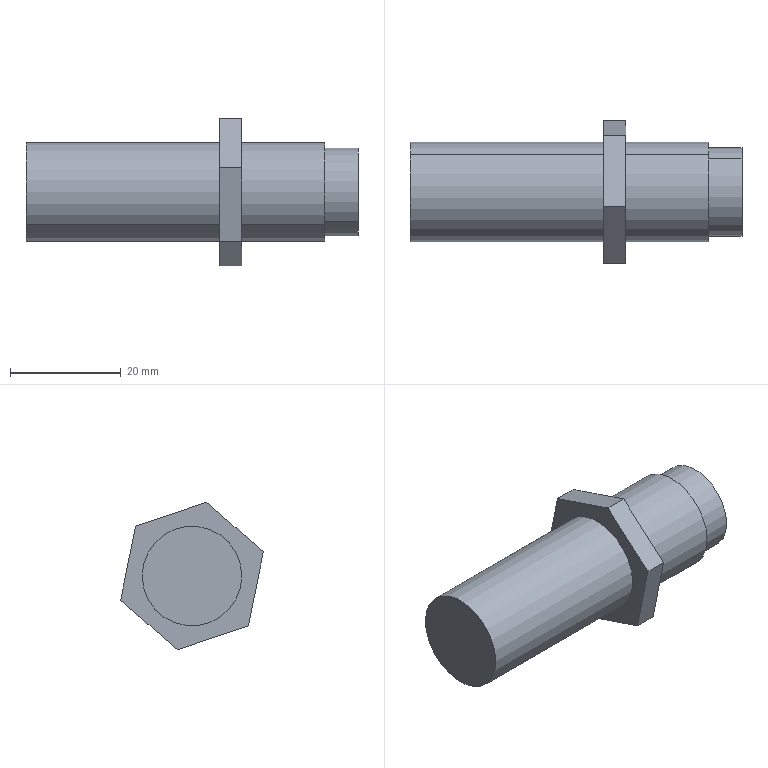Component | SolidWorks | M18GRYPQ-1 | 1 solid | 17 faces | box 60 x 25.76 x 26.67 mm | volume 15852 mm3 | plane 11 | cylinder 6 | commonest cylinder face diameters 18 x4 16 x2 | material 45
STEP:
#1=CARTESIAN_POINT('',(5.394,30.463,-5.396));
#2=VERTEX_POINT('',#1);
#3=CARTESIAN_POINT('',(5.394,29.931,-5.864));
#4=VERTEX_POINT('',#3);
#5=CARTESIAN_POINT('',(5.394,30.197,-5.63));
#6=DIRECTION('',(-1.,0.,0.));
#7=DIRECTION('',(0.,0.7513,0.6599));
#8=AXIS2_PLACEMENT_3D('',#5,#6,#7);
#9=CIRCLE('',#8,0.3543);
#10=EDGE_CURVE('',#2,#4,#9,.T.);
#11=ORIENTED_EDGE('',*,*,#10,.F.);
#12=CARTESIAN_POINT('',(6.772,30.463,-5.396));
#13=VERTEX_POINT('',#12);
#14=CARTESIAN_POINT('',(5.394,30.463,-5.396));
#15=DIRECTION('',(1.,-0.,-0.));
#16=VECTOR('',#15,39.37);
#17=LINE('',#14,#16);
#18=EDGE_CURVE('',#2,#13,#17,.T.);
#19=ORIENTED_EDGE('',*,*,#18,.T.);
#20=CARTESIAN_POINT('',(6.772,29.931,-5.864));
#21=VERTEX_POINT('',#20);
#22=CARTESIAN_POINT('',(6.772,30.197,-5.63));
#23=DIRECTION('',(1.,-0.,-0.));
#24=DIRECTION('',(0.,-0.7513,-0.6599));
#25=AXIS2_PLACEMENT_3D('',#22,#23,#24);
#26=CIRCLE('',#25,0.3543);
#27=EDGE_CURVE('',#21,#13,#26,.T.);
#28=ORIENTED_EDGE('',*,*,#27,.F.);
#29=CARTESIAN_POINT('',(5.394,29.931,-5.864));
#30=DIRECTION('',(1.,-0.,-0.));
#31=VECTOR('',#30,39.37);
#32=LINE('',#29,#31);
#33=EDGE_CURVE('',#4,#21,#32,.T.);
#34=ORIENTED_EDGE('',*,*,#33,.F.);
#35=EDGE_LOOP('',(#11,#19,#28,#34));
#36=FACE_OUTER_BOUND('',#35,.T.);
#37=CARTESIAN_POINT('',(5.394,30.197,-5.63));
#38=DIRECTION('',(1.,-0.,-0.));
#39=DIRECTION('',(0.,-0.7513,-0.6599));
#40=AXIS2_PLACEMENT_3D('',#37,#38,#39);
#41=CYLINDRICAL_SURFACE('',#40,0.3543);
#42=ADVANCED_FACE('',(#36),#41,.T.);
#43=CARTESIAN_POINT('',(6.929,29.931,-5.864));
#44=VERTEX_POINT('',#43);
#45=CARTESIAN_POINT('',(6.929,30.463,-5.396));
#46=VERTEX_POINT('',#45);
#47=CARTESIAN_POINT('',(6.929,30.197,-5.63));
#48=DIRECTION('',(1.,-0.,-0.));
#49=DIRECTION('',(0.,-0.7513,-0.6599));
#50=AXIS2_PLACEMENT_3D('',#47,#48,#49);
#51=CIRCLE('',#50,0.3543);
#52=EDGE_CURVE('',#44,#46,#51,.T.);
#53=ORIENTED_EDGE('',*,*,#52,.T.);
#54=CARTESIAN_POINT('',(7.52,30.463,-5.396));
#55=VERTEX_POINT('',#54);
#56=CARTESIAN_POINT('',(5.394,30.463,-5.396));
#57=DIRECTION('',(1.,-0.,-0.));
#58=VECTOR('',#57,39.37);
#59=LINE('',#56,#58);
#60=EDGE_CURVE('',#46,#55,#59,.T.);
#61=ORIENTED_EDGE('',*,*,#60,.T.);
#62=CARTESIAN_POINT('',(7.52,29.931,-5.864));
#63=VERTEX_POINT('',#62);
#64=CARTESIAN_POINT('',(7.52,30.197,-5.63));
#65=DIRECTION('',(-1.,0.,0.));
#66=DIRECTION('',(0.,0.7513,0.6599));
#67=AXIS2_PLACEMENT_3D('',#64,#65,#66);
#68=CIRCLE('',#67,0.3543);
#69=EDGE_CURVE('',#55,#63,#68,.T.);
#70=ORIENTED_EDGE('',*,*,#69,.T.);
#71=CARTESIAN_POINT('',(5.394,29.931,-5.864));
#72=DIRECTION('',(1.,-0.,-0.));
#73=VECTOR('',#72,39.37);
#74=LINE('',#71,#73);
#75=EDGE_CURVE('',#44,#63,#74,.T.);
#76=ORIENTED_EDGE('',*,*,#75,.F.);
#77=EDGE_LOOP('',(#53,#61,#70,#76));
#78=FACE_OUTER_BOUND('',#77,.T.);
#79=CARTESIAN_POINT('',(5.394,30.197,-5.63));
#80=DIRECTION('',(1.,-0.,-0.));
#81=DIRECTION('',(0.,-0.7513,-0.6599));
#82=AXIS2_PLACEMENT_3D('',#79,#80,#81);
#83=CYLINDRICAL_SURFACE('',#82,0.3543);
#84=ADVANCED_FACE('',(#78),#83,.T.);
#85=CARTESIAN_POINT('',(7.756,29.96,-5.838));
#86=VERTEX_POINT('',#85);
#87=CARTESIAN_POINT('',(7.756,30.433,-5.422));
#88=VERTEX_POINT('',#87);
#89=CARTESIAN_POINT('',(7.756,30.197,-5.63));
#90=DIRECTION('',(1.,-0.,-0.));
#91=DIRECTION('',(0.,-0.7513,-0.6599));
#92=AXIS2_PLACEMENT_3D('',#89,#90,#91);
#93=CIRCLE('',#92,0.315);
#94=EDGE_CURVE('',#86,#88,#93,.T.);
#95=ORIENTED_EDGE('',*,*,#94,.F.);
#96=CARTESIAN_POINT('',(7.52,29.96,-5.838));
#97=VERTEX_POINT('',#96);
#98=CARTESIAN_POINT('',(7.756,29.96,-5.838));
#99=DIRECTION('',(-1.,0.,0.));
#100=VECTOR('',#99,39.37);
#101=LINE('',#98,#100);
#102=EDGE_CURVE('',#86,#97,#101,.T.);
#103=ORIENTED_EDGE('',*,*,#102,.T.);
#104=CARTESIAN_POINT('',(7.52,30.433,-5.422));
#105=VERTEX_POINT('',#104);
#106=CARTESIAN_POINT('',(7.52,30.197,-5.63));
#107=DIRECTION('',(1.,-0.,-0.));
#108=DIRECTION('',(0.,-0.7513,-0.6599));
#109=AXIS2_PLACEMENT_3D('',#106,#107,#108);
#110=CIRCLE('',#109,0.315);
#111=EDGE_CURVE('',#97,#105,#110,.T.);
#112=ORIENTED_EDGE('',*,*,#111,.T.);
#113=CARTESIAN_POINT('',(7.756,30.433,-5.422));
#114=DIRECTION('',(-1.,0.,0.));
#115=VECTOR('',#114,39.37);
#116=LINE('',#113,#115);
#117=EDGE_CURVE('',#88,#105,#116,.T.);
#118=ORIENTED_EDGE('',*,*,#117,.F.);
#119=EDGE_LOOP('',(#95,#103,#112,#118));
#120=FACE_OUTER_BOUND('',#119,.T.);
#121=CARTESIAN_POINT('',(7.756,30.197,-5.63));
#122=DIRECTION('',(-1.,0.,0.));
#123=DIRECTION('',(0.,0.7513,0.6599));
#124=AXIS2_PLACEMENT_3D('',#121,#122,#123);
#125=CYLINDRICAL_SURFACE('',#124,0.315);
#126=ADVANCED_FACE('',(#120),#125,.T.);
#127=ORIENTED_EDGE('',*,*,#102,.F.);
#128=CARTESIAN_POINT('',(7.756,30.197,-5.63));
#129=DIRECTION('',(1.,-0.,-0.));
#130=DIRECTION('',(0.,-0.7513,-0.6599));
#131=AXIS2_PLACEMENT_3D('',#128,#129,#130);
#132=CIRCLE('',#131,0.315);
#133=EDGE_CURVE('',#88,#86,#132,.T.);
#134=ORIENTED_EDGE('',*,*,#133,.F.);
#135=ORIENTED_EDGE('',*,*,#117,.T.);
#136=CARTESIAN_POINT('',(7.52,30.197,-5.63));
#137=DIRECTION('',(1.,-0.,-0.));
#138=DIRECTION('',(0.,-0.7513,-0.6599));
#139=AXIS2_PLACEMENT_3D('',#136,#137,#138);
#140=CIRCLE('',#139,0.315);
#141=EDGE_CURVE('',#105,#97,#140,.T.);
#142=ORIENTED_EDGE('',*,*,#141,.T.);
#143=EDGE_LOOP('',(#127,#134,#135,#142));
#144=FACE_OUTER_BOUND('',#143,.T.);
#145=CARTESIAN_POINT('',(7.756,30.197,-5.63));
#146=DIRECTION('',(-1.,0.,0.));
#147=DIRECTION('',(0.,0.7513,0.6599));
#148=AXIS2_PLACEMENT_3D('',#145,#146,#147);
#149=CYLINDRICAL_SURFACE('',#148,0.315);
#150=ADVANCED_FACE('',(#144),#149,.T.);
#151=ORIENTED_EDGE('',*,*,#133,.T.);
#152=ORIENTED_EDGE('',*,*,#94,.T.);
#153=EDGE_LOOP('',(#151,#152));
#154=FACE_OUTER_BOUND('',#153,.T.);
#155=CARTESIAN_POINT('',(7.756,30.197,-5.63));
#156=DIRECTION('',(1.,-0.,-0.));
#157=DIRECTION('',(-0.,-0.7513,-0.6599));
#158=AXIS2_PLACEMENT_3D('',#155,#156,#157);
#159=PLANE('',#158);
#160=ADVANCED_FACE('',(#154),#159,.T.);
#161=ORIENTED_EDGE('',*,*,#60,.F.);
#162=CARTESIAN_POINT('',(6.929,30.197,-5.63));
#163=DIRECTION('',(1.,-0.,-0.));
#164=DIRECTION('',(0.,-0.7513,-0.6599));
#165=AXIS2_PLACEMENT_3D('',#162,#163,#164);
#166=CIRCLE('',#165,0.3543);
#167=EDGE_CURVE('',#46,#44,#166,.T.);
#168=ORIENTED_EDGE('',*,*,#167,.T.);
#169=ORIENTED_EDGE('',*,*,#75,.T.);
#170=CARTESIAN_POINT('',(7.52,30.197,-5.63));
#171=DIRECTION('',(-1.,0.,0.));
#172=DIRECTION('',(0.,0.7513,0.6599));
#173=AXIS2_PLACEMENT_3D('',#170,#171,#172);
#174=CIRCLE('',#173,0.3543);
#175=EDGE_CURVE('',#63,#55,#174,.T.);
#176=ORIENTED_EDGE('',*,*,#175,.T.);
#177=EDGE_LOOP('',(#161,#168,#169,#176));
#178=FACE_OUTER_BOUND('',#177,.T.);
#179=CARTESIAN_POINT('',(5.394,30.197,-5.63));
#180=DIRECTION('',(1.,-0.,-0.));
#181=DIRECTION('',(0.,-0.7513,-0.6599));
#182=AXIS2_PLACEMENT_3D('',#179,#180,#181);
#183=CYLINDRICAL_SURFACE('',#182,0.3543);
#184=ADVANCED_FACE('',(#178),#183,.T.);
#185=ORIENTED_EDGE('',*,*,#141,.F.);
#186=ORIENTED_EDGE('',*,*,#111,.F.);
#187=EDGE_LOOP('',(#185,#186));
#188=FACE_BOUND('',#187,.T.);
#189=ORIENTED_EDGE('',*,*,#175,.F.);
#190=ORIENTED_EDGE('',*,*,#69,.F.);
#191=EDGE_LOOP('',(#189,#190));
#192=FACE_OUTER_BOUND('',#191,.T.);
#193=CARTESIAN_POINT('',(7.52,30.197,-5.63));
#194=DIRECTION('',(-1.,0.,0.));
#195=DIRECTION('',(0.,0.7513,0.6599));
#196=AXIS2_PLACEMENT_3D('',#193,#194,#195);
#197=PLANE('',#196);
#198=ADVANCED_FACE('',(#188,#192),#197,.F.);
#199=CARTESIAN_POINT('',(6.929,29.69,-5.458));
#200=VERTEX_POINT('',#199);
#201=CARTESIAN_POINT('',(6.929,29.795,-5.983));
#202=VERTEX_POINT('',#201);
#203=CARTESIAN_POINT('',(6.929,29.69,-5.458));
#204=DIRECTION('',(-0.,0.1958,-0.9806));
#205=VECTOR('',#204,39.37);
#206=LINE('',#203,#205);
#207=EDGE_CURVE('',#200,#202,#206,.T.);
#208=ORIENTED_EDGE('',*,*,#207,.F.);
#209=CARTESIAN_POINT('',(6.772,29.69,-5.458));
#210=VERTEX_POINT('',#209);
#211=CARTESIAN_POINT('',(6.772,29.69,-5.458));
#212=DIRECTION('',(1.,-0.,-0.));
#213=VECTOR('',#212,39.37);
#214=LINE('',#211,#213);
#215=EDGE_CURVE('',#210,#200,#214,.T.);
#216=ORIENTED_EDGE('',*,*,#215,.F.);
#217=CARTESIAN_POINT('',(6.772,29.795,-5.983));
#218=VERTEX_POINT('',#217);
#219=CARTESIAN_POINT('',(6.772,29.69,-5.458));
#220=DIRECTION('',(-0.,0.1958,-0.9806));
#221=VECTOR('',#220,39.37);
#222=LINE('',#219,#221);
#223=EDGE_CURVE('',#210,#218,#222,.T.);
#224=ORIENTED_EDGE('',*,*,#223,.T.);
#225=CARTESIAN_POINT('',(6.772,29.795,-5.983));
#226=DIRECTION('',(1.,-0.,-0.));
#227=VECTOR('',#226,39.37);
#228=LINE('',#225,#227);
#229=EDGE_CURVE('',#218,#202,#228,.T.);
#230=ORIENTED_EDGE('',*,*,#229,.T.);
#231=EDGE_LOOP('',(#208,#216,#224,#230));
#232=FACE_OUTER_BOUND('',#231,.T.);
#233=CARTESIAN_POINT('',(6.772,29.69,-5.458));
#234=DIRECTION('',(-0.,-0.9806,-0.1958));
#235=DIRECTION('',(-0.,0.1958,-0.9806));
#236=AXIS2_PLACEMENT_3D('',#233,#234,#235);
#237=PLANE('',#236);
#238=ADVANCED_FACE('',(#232),#237,.T.);
#239=CARTESIAN_POINT('',(6.929,30.092,-5.105));
#240=VERTEX_POINT('',#239);
#241=CARTESIAN_POINT('',(6.929,30.092,-5.105));
#242=DIRECTION('',(-0.,-0.7513,-0.6599));
#243=VECTOR('',#242,39.37);
#244=LINE('',#241,#243);
#245=EDGE_CURVE('',#240,#200,#244,.T.);
#246=ORIENTED_EDGE('',*,*,#245,.F.);
#247=CARTESIAN_POINT('',(6.772,30.092,-5.105));
#248=VERTEX_POINT('',#247);
#249=CARTESIAN_POINT('',(6.772,30.092,-5.105));
#250=DIRECTION('',(1.,-0.,-0.));
#251=VECTOR('',#250,39.37);
#252=LINE('',#249,#251);
#253=EDGE_CURVE('',#248,#240,#252,.T.);
#254=ORIENTED_EDGE('',*,*,#253,.F.);
#255=CARTESIAN_POINT('',(6.772,30.092,-5.105));
#256=DIRECTION('',(-0.,-0.7513,-0.6599));
#257=VECTOR('',#256,39.37);
#258=LINE('',#255,#257);
#259=EDGE_CURVE('',#248,#210,#258,.T.);
#260=ORIENTED_EDGE('',*,*,#259,.T.);
#261=ORIENTED_EDGE('',*,*,#215,.T.);
#262=EDGE_LOOP('',(#246,#254,#260,#261));
#263=FACE_OUTER_BOUND('',#262,.T.);
#264=CARTESIAN_POINT('',(6.772,30.092,-5.105));
#265=DIRECTION('',(-0.,-0.6599,0.7513));
#266=DIRECTION('',(-0.,-0.7513,-0.6599));
#267=AXIS2_PLACEMENT_3D('',#264,#265,#266);
#268=PLANE('',#267);
#269=ADVANCED_FACE('',(#263),#268,.T.);
#270=CARTESIAN_POINT('',(6.929,30.599,-5.277));
#271=VERTEX_POINT('',#270);
#272=CARTESIAN_POINT('',(6.929,30.599,-5.277));
#273=DIRECTION('',(-0.,-0.9472,0.3207));
#274=VECTOR('',#273,39.37);
#275=LINE('',#272,#274);
#276=EDGE_CURVE('',#271,#240,#275,.T.);
#277=ORIENTED_EDGE('',*,*,#276,.F.);
#278=CARTESIAN_POINT('',(6.772,30.599,-5.277));
#279=VERTEX_POINT('',#278);
#280=CARTESIAN_POINT('',(6.772,30.599,-5.277));
#281=DIRECTION('',(1.,-0.,-0.));
#282=VECTOR('',#281,39.37);
#283=LINE('',#280,#282);
#284=EDGE_CURVE('',#279,#271,#283,.T.);
#285=ORIENTED_EDGE('',*,*,#284,.F.);
#286=CARTESIAN_POINT('',(6.772,30.599,-5.277));
#287=DIRECTION('',(-0.,-0.9472,0.3207));
#288=VECTOR('',#287,39.37);
#289=LINE('',#286,#288);
#290=EDGE_CURVE('',#279,#248,#289,.T.);
#291=ORIENTED_EDGE('',*,*,#290,.T.);
#292=ORIENTED_EDGE('',*,*,#253,.T.);
#293=EDGE_LOOP('',(#277,#285,#291,#292));
#294=FACE_OUTER_BOUND('',#293,.T.);
#295=CARTESIAN_POINT('',(6.772,30.599,-5.277));
#296=DIRECTION('',(0.,0.3207,0.9472));
#297=DIRECTION('',(-0.,-0.9472,0.3207));
#298=AXIS2_PLACEMENT_3D('',#295,#296,#297);
#299=PLANE('',#298);
#300=ADVANCED_FACE('',(#294),#299,.T.);
#301=CARTESIAN_POINT('',(6.929,30.704,-5.802));
#302=VERTEX_POINT('',#301);
#303=CARTESIAN_POINT('',(6.929,30.704,-5.802));
#304=DIRECTION('',(0.,-0.1958,0.9806));
#305=VECTOR('',#304,39.37);
#306=LINE('',#303,#305);
#307=EDGE_CURVE('',#302,#271,#306,.T.);
#308=ORIENTED_EDGE('',*,*,#307,.F.);
#309=CARTESIAN_POINT('',(6.772,30.704,-5.802));
#310=VERTEX_POINT('',#309);
#311=CARTESIAN_POINT('',(6.772,30.704,-5.802));
#312=DIRECTION('',(1.,-0.,-0.));
#313=VECTOR('',#312,39.37);
#314=LINE('',#311,#313);
#315=EDGE_CURVE('',#310,#302,#314,.T.);
#316=ORIENTED_EDGE('',*,*,#315,.F.);
#317=CARTESIAN_POINT('',(6.772,30.704,-5.802));
#318=DIRECTION('',(0.,-0.1958,0.9806));
#319=VECTOR('',#318,39.37);
#320=LINE('',#317,#319);
#321=EDGE_CURVE('',#310,#279,#320,.T.);
#322=ORIENTED_EDGE('',*,*,#321,.T.);
#323=ORIENTED_EDGE('',*,*,#284,.T.);
#324=EDGE_LOOP('',(#308,#316,#322,#323));
#325=FACE_OUTER_BOUND('',#324,.T.);
#326=CARTESIAN_POINT('',(6.772,30.704,-5.802));
#327=DIRECTION('',(0.,0.9806,0.1958));
#328=DIRECTION('',(0.,-0.1958,0.9806));
#329=AXIS2_PLACEMENT_3D('',#326,#327,#328);
#330=PLANE('',#329);
#331=ADVANCED_FACE('',(#325),#330,.T.);
#332=CARTESIAN_POINT('',(6.929,30.302,-6.155));
#333=VERTEX_POINT('',#332);
#334=CARTESIAN_POINT('',(6.929,30.302,-6.155));
#335=DIRECTION('',(0.,0.7513,0.6599));
#336=VECTOR('',#335,39.37);
#337=LINE('',#334,#336);
#338=EDGE_CURVE('',#333,#302,#337,.T.);
#339=ORIENTED_EDGE('',*,*,#338,.F.);
#340=CARTESIAN_POINT('',(6.772,30.302,-6.155));
#341=VERTEX_POINT('',#340);
#342=CARTESIAN_POINT('',(6.772,30.302,-6.155));
#343=DIRECTION('',(1.,-0.,-0.));
#344=VECTOR('',#343,39.37);
#345=LINE('',#342,#344);
#346=EDGE_CURVE('',#341,#333,#345,.T.);
#347=ORIENTED_EDGE('',*,*,#346,.F.);
#348=CARTESIAN_POINT('',(6.772,30.302,-6.155));
#349=DIRECTION('',(0.,0.7513,0.6599));
#350=VECTOR('',#349,39.37);
#351=LINE('',#348,#350);
#352=EDGE_CURVE('',#341,#310,#351,.T.);
#353=ORIENTED_EDGE('',*,*,#352,.T.);
#354=ORIENTED_EDGE('',*,*,#315,.T.);
#355=EDGE_LOOP('',(#339,#347,#353,#354));
#356=FACE_OUTER_BOUND('',#355,.T.);
#357=CARTESIAN_POINT('',(6.772,30.302,-6.155));
#358=DIRECTION('',(0.,0.6599,-0.7513));
#359=DIRECTION('',(1.,-0.,-0.));
#360=AXIS2_PLACEMENT_3D('',#357,#358,#359);
#361=PLANE('',#360);
#362=ADVANCED_FACE('',(#356),#361,.T.);
#363=CARTESIAN_POINT('',(6.929,29.795,-5.983));
#364=DIRECTION('',(0.,0.9472,-0.3207));
#365=VECTOR('',#364,39.37);
#366=LINE('',#363,#365);
#367=EDGE_CURVE('',#202,#333,#366,.T.);
#368=ORIENTED_EDGE('',*,*,#367,.F.);
#369=ORIENTED_EDGE('',*,*,#229,.F.);
#370=CARTESIAN_POINT('',(6.772,29.795,-5.983));
#371=DIRECTION('',(0.,0.9472,-0.3207));
#372=VECTOR('',#371,39.37);
#373=LINE('',#370,#372);
#374=EDGE_CURVE('',#218,#341,#373,.T.);
#375=ORIENTED_EDGE('',*,*,#374,.T.);
#376=ORIENTED_EDGE('',*,*,#346,.T.);
#377=EDGE_LOOP('',(#368,#369,#375,#376));
#378=FACE_OUTER_BOUND('',#377,.T.);
#379=CARTESIAN_POINT('',(6.772,29.795,-5.983));
#380=DIRECTION('',(-0.,-0.3207,-0.9472));
#381=DIRECTION('',(0.,0.9472,-0.3207));
#382=AXIS2_PLACEMENT_3D('',#379,#380,#381);
#383=PLANE('',#382);
#384=ADVANCED_FACE('',(#378),#383,.T.);
#385=ORIENTED_EDGE('',*,*,#27,.T.);
#386=CARTESIAN_POINT('',(6.772,30.197,-5.63));
#387=DIRECTION('',(1.,-0.,-0.));
#388=DIRECTION('',(0.,-0.7513,-0.6599));
#389=AXIS2_PLACEMENT_3D('',#386,#387,#388);
#390=CIRCLE('',#389,0.3543);
#391=EDGE_CURVE('',#13,#21,#390,.T.);
#392=ORIENTED_EDGE('',*,*,#391,.T.);
#393=EDGE_LOOP('',(#385,#392));
#394=FACE_BOUND('',#393,.T.);
#395=ORIENTED_EDGE('',*,*,#223,.F.);
#396=ORIENTED_EDGE('',*,*,#259,.F.);
#397=ORIENTED_EDGE('',*,*,#290,.F.);
#398=ORIENTED_EDGE('',*,*,#321,.F.);
#399=ORIENTED_EDGE('',*,*,#352,.F.);
#400=ORIENTED_EDGE('',*,*,#374,.F.);
#401=EDGE_LOOP('',(#395,#396,#397,#398,#399,#400));
#402=FACE_OUTER_BOUND('',#401,.T.);
#403=CARTESIAN_POINT('',(6.772,30.197,-5.63));
#404=DIRECTION('',(1.,-0.,-0.));
#405=DIRECTION('',(-0.,-0.7513,-0.6599));
#406=AXIS2_PLACEMENT_3D('',#403,#404,#405);
#407=PLANE('',#406);
#408=ADVANCED_FACE('',(#394,#402),#407,.F.);
#409=ORIENTED_EDGE('',*,*,#52,.F.);
#410=ORIENTED_EDGE('',*,*,#167,.F.);
#411=EDGE_LOOP('',(#409,#410));
#412=FACE_BOUND('',#411,.T.);
#413=ORIENTED_EDGE('',*,*,#207,.T.);
#414=ORIENTED_EDGE('',*,*,#367,.T.);
#415=ORIENTED_EDGE('',*,*,#338,.T.);
#416=ORIENTED_EDGE('',*,*,#307,.T.);
#417=ORIENTED_EDGE('',*,*,#276,.T.);
#418=ORIENTED_EDGE('',*,*,#245,.T.);
#419=EDGE_LOOP('',(#413,#414,#415,#416,#417,#418));
#420=FACE_OUTER_BOUND('',#419,.T.);
#421=CARTESIAN_POINT('',(6.929,30.197,-5.63));
#422=DIRECTION('',(1.,-0.,-0.));
#423=DIRECTION('',(-0.,-0.7513,-0.6599));
#424=AXIS2_PLACEMENT_3D('',#421,#422,#423);
#425=PLANE('',#424);
#426=ADVANCED_FACE('',(#412,#420),#425,.T.);
#427=CARTESIAN_POINT('',(5.394,30.197,-5.63));
#428=DIRECTION('',(-1.,0.,0.));
#429=DIRECTION('',(0.,0.7513,0.6599));
#430=AXIS2_PLACEMENT_3D('',#427,#428,#429);
#431=CIRCLE('',#430,0.3543);
#432=EDGE_CURVE('',#4,#2,#431,.T.);
#433=ORIENTED_EDGE('',*,*,#432,.T.);
#434=ORIENTED_EDGE('',*,*,#10,.T.);
#435=EDGE_LOOP('',(#433,#434));
#436=FACE_OUTER_BOUND('',#435,.T.);
#437=CARTESIAN_POINT('',(5.394,30.197,-5.63));
#438=DIRECTION('',(-1.,0.,0.));
#439=DIRECTION('',(0.,0.7513,0.6599));
#440=AXIS2_PLACEMENT_3D('',#437,#438,#439);
#441=PLANE('',#440);
#442=ADVANCED_FACE('',(#436),#441,.T.);
#443=ORIENTED_EDGE('',*,*,#18,.F.);
#444=ORIENTED_EDGE('',*,*,#432,.F.);
#445=ORIENTED_EDGE('',*,*,#33,.T.);
#446=ORIENTED_EDGE('',*,*,#391,.F.);
#447=EDGE_LOOP('',(#443,#444,#445,#446));
#448=FACE_OUTER_BOUND('',#447,.T.);
#449=CARTESIAN_POINT('',(5.394,30.197,-5.63));
#450=DIRECTION('',(1.,-0.,-0.));
#451=DIRECTION('',(0.,-0.7513,-0.6599));
#452=AXIS2_PLACEMENT_3D('',#449,#450,#451);
#453=CYLINDRICAL_SURFACE('',#452,0.3543);
#454=ADVANCED_FACE('',(#448),#453,.T.);
#455=CLOSED_SHELL('',(#42,#84,#126,#150,#160,#184,#198,#238,#269,#300,#331,#362,#384,#408,#426,#442,#454));
#456=MANIFOLD_SOLID_BREP('',#455);
#457=CARTESIAN_POINT('',(0.,0.,0.));
#458=DIRECTION('',(0.,0.,1.));
#459=DIRECTION('',(1.,0.,0.));
#460=AXIS2_PLACEMENT_3D('',#457,#458,#459);
#461=(LENGTH_UNIT()NAMED_UNIT(*)SI_UNIT($,.METRE.));
#462=LENGTH_MEASURE_WITH_UNIT(LENGTH_MEASURE(0.0254),#461);
#463=DIMENSIONAL_EXPONENTS(1.,0.,0.,0.,0.,0.,0.);
#464=(CONVERSION_BASED_UNIT('',#462)LENGTH_UNIT()NAMED_UNIT(#463));
#465=UNCERTAINTY_MEASURE_WITH_UNIT(LENGTH_MEASURE(0.00001),#464,'','');
#466=(NAMED_UNIT(*)PLANE_ANGLE_UNIT()SI_UNIT($,.RADIAN.));
#467=(NAMED_UNIT(*)SI_UNIT($,.STERADIAN.)SOLID_ANGLE_UNIT());
#468=(GEOMETRIC_REPRESENTATION_CONTEXT(3)GLOBAL_UNCERTAINTY_ASSIGNED_CONTEXT((#465))GLOBAL_UNIT_ASSIGNED_CONTEXT((#464,#466,#467))REPRESENTATION_CONTEXT('',''));
#469=ADVANCED_BREP_SHAPE_REPRESENTATION('',(#456,#460),#468);
#470=COLOUR_RGB('',0.7922,0.8196,0.9333);
#471=FILL_AREA_STYLE_COLOUR('',#470);
#472=FILL_AREA_STYLE('',(#471));
#473=SURFACE_STYLE_FILL_AREA(#472);
#474=SURFACE_SIDE_STYLE('',(#473));
#475=SURFACE_STYLE_USAGE(.BOTH.,#474);
#476=PRESENTATION_STYLE_ASSIGNMENT((#475));
#477=STYLED_ITEM('',(#476),#456);
#478=(LENGTH_UNIT()NAMED_UNIT(*)SI_UNIT($,.METRE.));
#479=LENGTH_MEASURE_WITH_UNIT(LENGTH_MEASURE(0.0254),#478);
#480=DIMENSIONAL_EXPONENTS(1.,0.,0.,0.,0.,0.,0.);
#481=(CONVERSION_BASED_UNIT('',#479)LENGTH_UNIT()NAMED_UNIT(#480));
#482=UNCERTAINTY_MEASURE_WITH_UNIT(LENGTH_MEASURE(0.00001),#481,'','');
#483=(NAMED_UNIT(*)PLANE_ANGLE_UNIT()SI_UNIT($,.RADIAN.));
#484=(NAMED_UNIT(*)SI_UNIT($,.STERADIAN.)SOLID_ANGLE_UNIT());
#485=(GEOMETRIC_REPRESENTATION_CONTEXT(3)GLOBAL_UNCERTAINTY_ASSIGNED_CONTEXT((#482))GLOBAL_UNIT_ASSIGNED_CONTEXT((#481,#483,#484))REPRESENTATION_CONTEXT('',''));
#486=MECHANICAL_DESIGN_GEOMETRIC_PRESENTATION_REPRESENTATION('',(#477),#485);
#487=PRESENTATION_LAYER_ASSIGNMENT('','',(#477));